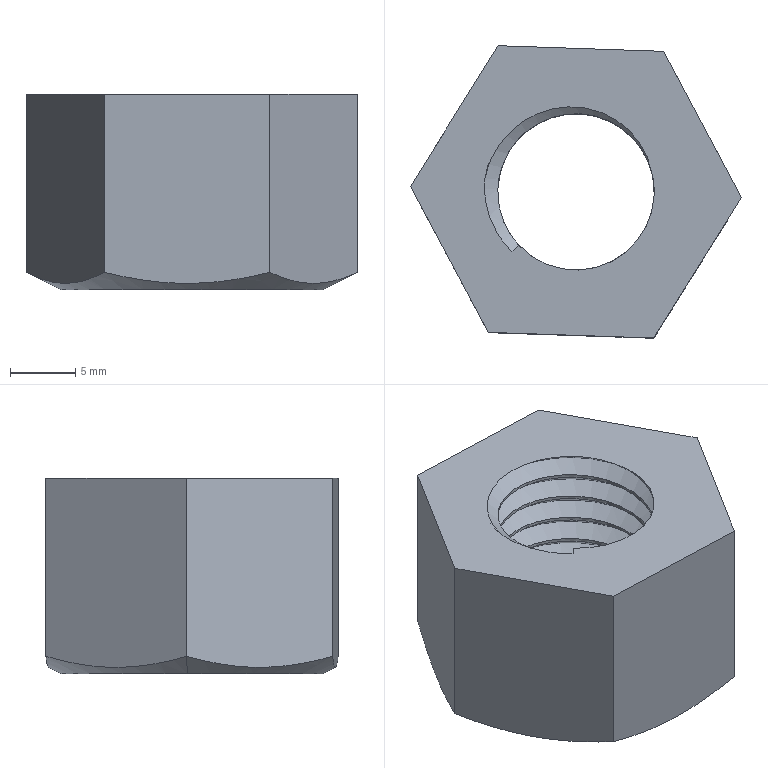Component | SolidWorks | GussetPlateAssembly-1_Nut-1 | 1 solid | 31 faces | volume 4267 mm3 | cylinder 17 | plane 10 | cone 2 | spline 2 | commonest cylinder face diameters 12 x17